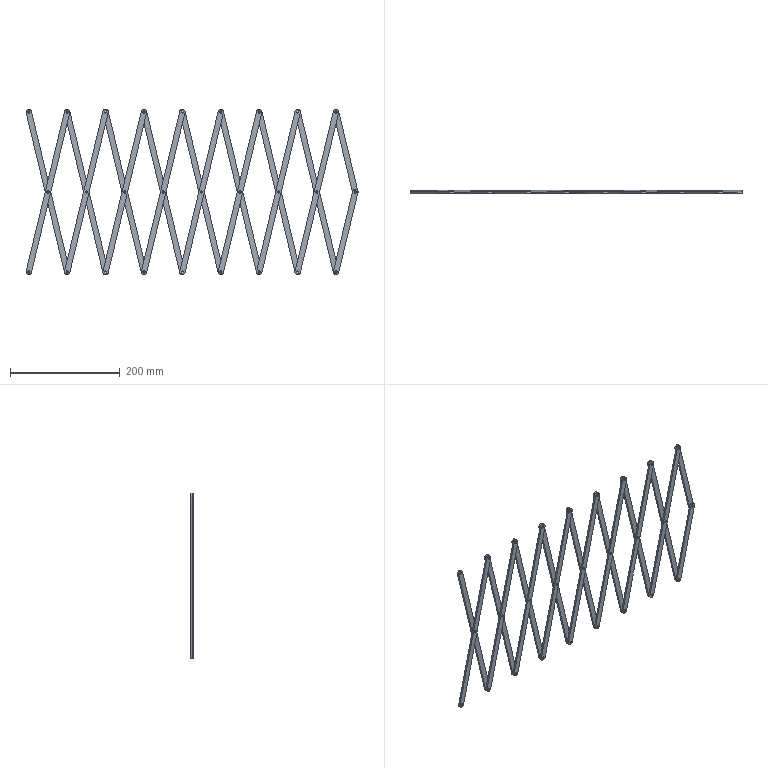Component | NX | MIRROR_SCISSOR_ROD | 18 solids | 160 faces | volume 155281 mm3 | cylinder 88 | plane 72 | commonest cylinder face diameters 4 x52 10 x36